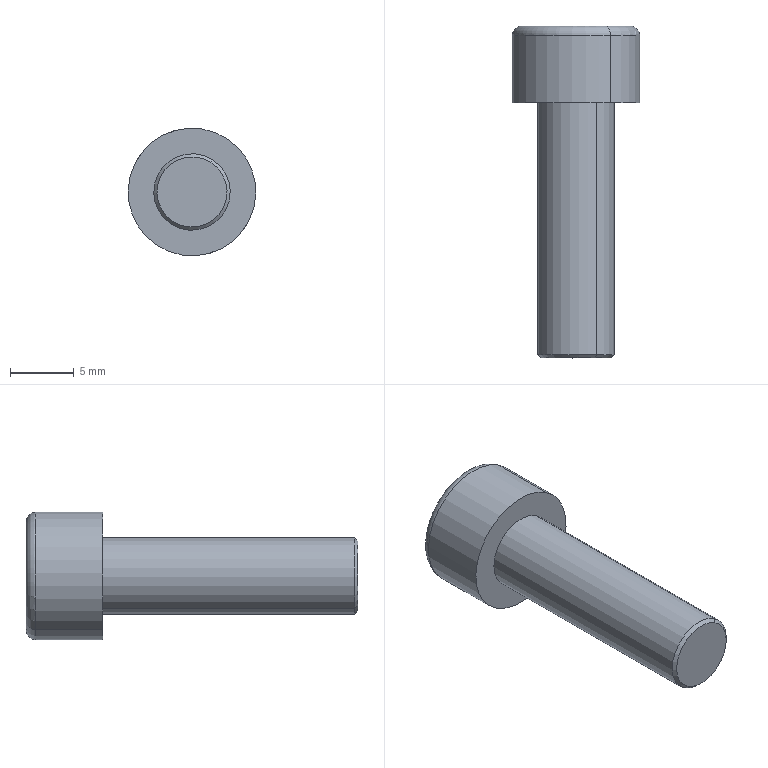Component | SolidWorks | hexagon socket head cap screws gb-17 | 1 solid | 25 faces | box 10 x 26 x 10 mm | volume 958 mm3 | plane 15 | cone 4 | cylinder 4 | torus 2 | commonest cylinder face diameters 6 x2 10 x2
STEP:
#1=COLOUR_RGB('',0.7922,0.8196,0.9333);
#2=FILL_AREA_STYLE_COLOUR('',#1);
#3=FILL_AREA_STYLE('',(#2));
#4=SURFACE_STYLE_FILL_AREA(#3);
#5=SURFACE_SIDE_STYLE('',(#4));
#6=SURFACE_STYLE_USAGE(.BOTH.,#5);
#7=PRESENTATION_STYLE_ASSIGNMENT((#6));
#8=CARTESIAN_POINT('',(-4.388,20.52,21.251));
#9=VERTEX_POINT('',#8);
#10=CARTESIAN_POINT('',(-4.271,20.52,21.433));
#11=VERTEX_POINT('',#10);
#12=CARTESIAN_POINT('',(-4.33,20.52,21.342));
#13=DIRECTION('',(0.,-1.,0.));
#14=DIRECTION('',(-0.5407,0.,-0.8412));
#15=AXIS2_PLACEMENT_3D('',#12,#13,#14);
#16=CIRCLE('',#15,0.1083);
#17=EDGE_CURVE('',#9,#11,#16,.T.);
#18=ORIENTED_EDGE('',*,*,#17,.F.);
#19=CARTESIAN_POINT('',(-4.394,20.53,21.243));
#20=VERTEX_POINT('',#19);
#21=CARTESIAN_POINT('',(-4.388,20.52,21.251));
#22=DIRECTION('',(-0.3823,0.7071,-0.5948));
#23=VECTOR('',#22,39.37);
#24=LINE('',#21,#23);
#25=EDGE_CURVE('',#9,#20,#24,.T.);
#26=ORIENTED_EDGE('',*,*,#25,.T.);
#27=CARTESIAN_POINT('',(-4.266,20.53,21.441));
#28=VERTEX_POINT('',#27);
#29=CARTESIAN_POINT('',(-4.33,20.53,21.342));
#30=DIRECTION('',(0.,1.,0.));
#31=DIRECTION('',(-0.5407,0.,-0.8412));
#32=AXIS2_PLACEMENT_3D('',#29,#30,#31);
#33=CIRCLE('',#32,0.1181);
#34=EDGE_CURVE('',#28,#20,#33,.T.);
#35=ORIENTED_EDGE('',*,*,#34,.F.);
#36=CARTESIAN_POINT('',(-4.271,20.52,21.433));
#37=DIRECTION('',(0.3823,0.7071,0.5948));
#38=VECTOR('',#37,39.37);
#39=LINE('',#36,#38);
#40=EDGE_CURVE('',#11,#28,#39,.T.);
#41=ORIENTED_EDGE('',*,*,#40,.F.);
#42=EDGE_LOOP('',(#18,#26,#35,#41));
#43=FACE_OUTER_BOUND('',#42,.T.);
#44=CARTESIAN_POINT('',(-4.33,20.52,21.342));
#45=DIRECTION('',(0.,1.,0.));
#46=DIRECTION('',(0.5407,0.,0.8412));
#47=AXIS2_PLACEMENT_3D('',#44,#45,#46);
#48=CONICAL_SURFACE('',#47,0.1083,0.7854);
#49=ADVANCED_FACE('',(#43),#48,.T.);
#50=CARTESIAN_POINT('',(-4.239,21.544,21.483));
#51=VERTEX_POINT('',#50);
#52=CARTESIAN_POINT('',(-4.42,21.544,21.201));
#53=VERTEX_POINT('',#52);
#54=CARTESIAN_POINT('',(-4.33,21.544,21.342));
#55=DIRECTION('',(0.,1.,0.));
#56=DIRECTION('',(-0.5407,0.,-0.8412));
#57=AXIS2_PLACEMENT_3D('',#54,#55,#56);
#58=CIRCLE('',#57,0.1673);
#59=EDGE_CURVE('',#51,#53,#58,.T.);
#60=ORIENTED_EDGE('',*,*,#59,.F.);
#61=CARTESIAN_POINT('',(-4.223,21.515,21.508));
#62=VERTEX_POINT('',#61);
#63=CARTESIAN_POINT('',(-4.239,21.515,21.483));
#64=DIRECTION('',(0.8412,0.,-0.5407));
#65=DIRECTION('',(-0.5407,0.,-0.8412));
#66=AXIS2_PLACEMENT_3D('',#63,#64,#65);
#67=CIRCLE('',#66,0.02953);
#68=EDGE_CURVE('',#51,#62,#67,.T.);
#69=ORIENTED_EDGE('',*,*,#68,.T.);
#70=CARTESIAN_POINT('',(-4.436,21.515,21.176));
#71=VERTEX_POINT('',#70);
#72=CARTESIAN_POINT('',(-4.33,21.515,21.342));
#73=DIRECTION('',(0.,-1.,0.));
#74=DIRECTION('',(-0.5407,0.,-0.8412));
#75=AXIS2_PLACEMENT_3D('',#72,#73,#74);
#76=CIRCLE('',#75,0.1969);
#77=EDGE_CURVE('',#71,#62,#76,.T.);
#78=ORIENTED_EDGE('',*,*,#77,.F.);
#79=CARTESIAN_POINT('',(-4.42,21.515,21.201));
#80=DIRECTION('',(-0.8412,0.,0.5407));
#81=DIRECTION('',(0.5407,0.,0.8412));
#82=AXIS2_PLACEMENT_3D('',#79,#80,#81);
#83=CIRCLE('',#82,0.02953);
#84=EDGE_CURVE('',#53,#71,#83,.T.);
#85=ORIENTED_EDGE('',*,*,#84,.F.);
#86=EDGE_LOOP('',(#60,#69,#78,#85));
#87=FACE_OUTER_BOUND('',#86,.T.);
#88=CARTESIAN_POINT('',(-4.33,21.515,21.342));
#89=DIRECTION('',(0.,-1.,0.));
#90=DIRECTION('',(-0.5407,0.,-0.8412));
#91=AXIS2_PLACEMENT_3D('',#88,#89,#90);
#92=TOROIDAL_SURFACE('',#91,0.1673,0.02953);
#93=ADVANCED_FACE('',(#87),#92,.T.);
#94=CARTESIAN_POINT('',(-4.33,21.369,21.342));
#95=VERTEX_POINT('',#94);
#96=CARTESIAN_POINT('',(-4.276,21.426,21.425));
#97=VERTEX_POINT('',#96);
#98=CARTESIAN_POINT('',(-4.276,21.426,21.425));
#99=DIRECTION('',(0.4682,0.5,0.7285));
#100=VECTOR('',#99,39.37);
#101=LINE('',#98,#100);
#102=EDGE_CURVE('',#95,#97,#101,.T.);
#103=ORIENTED_EDGE('',*,*,#102,.F.);
#104=CARTESIAN_POINT('',(-4.383,21.426,21.259));
#105=VERTEX_POINT('',#104);
#106=CARTESIAN_POINT('',(-4.383,21.426,21.259));
#107=DIRECTION('',(-0.4682,0.5,-0.7285));
#108=VECTOR('',#107,39.37);
#109=LINE('',#106,#108);
#110=EDGE_CURVE('',#95,#105,#109,.T.);
#111=ORIENTED_EDGE('',*,*,#110,.T.);
#112=CARTESIAN_POINT('',(-4.417,21.426,21.297));
#113=VERTEX_POINT('',#112);
#114=CARTESIAN_POINT('',(-4.33,21.426,21.342));
#115=DIRECTION('',(0.,1.,0.));
#116=DIRECTION('',(-0.5407,0.,-0.8412));
#117=AXIS2_PLACEMENT_3D('',#114,#115,#116);
#118=CIRCLE('',#117,0.09843);
#119=EDGE_CURVE('',#105,#113,#118,.T.);
#120=ORIENTED_EDGE('',*,*,#119,.T.);
#121=CARTESIAN_POINT('',(-4.413,21.426,21.395));
#122=VERTEX_POINT('',#121);
#123=CARTESIAN_POINT('',(-4.33,21.426,21.342));
#124=DIRECTION('',(0.,1.,0.));
#125=DIRECTION('',(-0.5407,0.,-0.8412));
#126=AXIS2_PLACEMENT_3D('',#123,#124,#125);
#127=CIRCLE('',#126,0.09843);
#128=EDGE_CURVE('',#113,#122,#127,.T.);
#129=ORIENTED_EDGE('',*,*,#128,.T.);
#130=CARTESIAN_POINT('',(-4.325,21.426,21.44));
#131=VERTEX_POINT('',#130);
#132=CARTESIAN_POINT('',(-4.33,21.426,21.342));
#133=DIRECTION('',(0.,1.,0.));
#134=DIRECTION('',(-0.5407,0.,-0.8412));
#135=AXIS2_PLACEMENT_3D('',#132,#133,#134);
#136=CIRCLE('',#135,0.09843);
#137=EDGE_CURVE('',#122,#131,#136,.T.);
#138=ORIENTED_EDGE('',*,*,#137,.T.);
#139=CARTESIAN_POINT('',(-4.33,21.426,21.342));
#140=DIRECTION('',(0.,1.,0.));
#141=DIRECTION('',(-0.5407,0.,-0.8412));
#142=AXIS2_PLACEMENT_3D('',#139,#140,#141);
#143=CIRCLE('',#142,0.09843);
#144=EDGE_CURVE('',#131,#97,#143,.T.);
#145=ORIENTED_EDGE('',*,*,#144,.T.);
#146=EDGE_LOOP('',(#103,#111,#120,#129,#138,#145));
#147=FACE_OUTER_BOUND('',#146,.T.);
#148=CARTESIAN_POINT('',(-4.33,21.426,21.342));
#149=DIRECTION('',(0.,1.,0.));
#150=DIRECTION('',(0.5407,0.,0.8412));
#151=AXIS2_PLACEMENT_3D('',#148,#149,#150);
#152=CONICAL_SURFACE('',#151,0.09843,1.047);
#153=ADVANCED_FACE('',(#147),#152,.F.);
#154=ORIENTED_EDGE('',*,*,#34,.T.);
#155=CARTESIAN_POINT('',(-4.394,21.308,21.243));
#156=VERTEX_POINT('',#155);
#157=CARTESIAN_POINT('',(-4.394,20.52,21.243));
#158=DIRECTION('',(0.,1.,0.));
#159=VECTOR('',#158,39.37);
#160=LINE('',#157,#159);
#161=EDGE_CURVE('',#20,#156,#160,.T.);
#162=ORIENTED_EDGE('',*,*,#161,.T.);
#163=CARTESIAN_POINT('',(-4.266,21.308,21.441));
#164=VERTEX_POINT('',#163);
#165=CARTESIAN_POINT('',(-4.33,21.308,21.342));
#166=DIRECTION('',(0.,-1.,0.));
#167=DIRECTION('',(-0.5407,0.,-0.8412));
#168=AXIS2_PLACEMENT_3D('',#165,#166,#167);
#169=CIRCLE('',#168,0.1181);
#170=EDGE_CURVE('',#156,#164,#169,.T.);
#171=ORIENTED_EDGE('',*,*,#170,.T.);
#172=CARTESIAN_POINT('',(-4.266,20.52,21.441));
#173=DIRECTION('',(0.,1.,0.));
#174=VECTOR('',#173,39.37);
#175=LINE('',#172,#174);
#176=EDGE_CURVE('',#28,#164,#175,.T.);
#177=ORIENTED_EDGE('',*,*,#176,.F.);
#178=EDGE_LOOP('',(#154,#162,#171,#177));
#179=FACE_OUTER_BOUND('',#178,.T.);
#180=CARTESIAN_POINT('',(-4.33,20.52,21.342));
#181=DIRECTION('',(0.,1.,0.));
#182=DIRECTION('',(0.5407,0.,0.8412));
#183=AXIS2_PLACEMENT_3D('',#180,#181,#182);
#184=CYLINDRICAL_SURFACE('',#183,0.1181);
#185=ADVANCED_FACE('',(#179),#184,.T.);
#186=CARTESIAN_POINT('',(-4.436,21.308,21.176));
#187=VERTEX_POINT('',#186);
#188=CARTESIAN_POINT('',(-4.223,21.308,21.508));
#189=VERTEX_POINT('',#188);
#190=CARTESIAN_POINT('',(-4.33,21.308,21.342));
#191=DIRECTION('',(0.,-1.,0.));
#192=DIRECTION('',(-0.5407,0.,-0.8412));
#193=AXIS2_PLACEMENT_3D('',#190,#191,#192);
#194=CIRCLE('',#193,0.1969);
#195=EDGE_CURVE('',#187,#189,#194,.T.);
#196=ORIENTED_EDGE('',*,*,#195,.F.);
#197=CARTESIAN_POINT('',(-4.436,21.308,21.176));
#198=DIRECTION('',(0.,1.,0.));
#199=VECTOR('',#198,39.37);
#200=LINE('',#197,#199);
#201=EDGE_CURVE('',#187,#71,#200,.T.);
#202=ORIENTED_EDGE('',*,*,#201,.T.);
#203=ORIENTED_EDGE('',*,*,#77,.T.);
#204=CARTESIAN_POINT('',(-4.223,21.308,21.508));
#205=DIRECTION('',(0.,1.,0.));
#206=VECTOR('',#205,39.37);
#207=LINE('',#204,#206);
#208=EDGE_CURVE('',#189,#62,#207,.T.);
#209=ORIENTED_EDGE('',*,*,#208,.F.);
#210=EDGE_LOOP('',(#196,#202,#203,#209));
#211=FACE_OUTER_BOUND('',#210,.T.);
#212=CARTESIAN_POINT('',(-4.33,21.308,21.342));
#213=DIRECTION('',(0.,1.,0.));
#214=DIRECTION('',(0.5407,0.,0.8412));
#215=AXIS2_PLACEMENT_3D('',#212,#213,#214);
#216=CYLINDRICAL_SURFACE('',#215,0.1969);
#217=ADVANCED_FACE('',(#211),#216,.T.);
#218=ORIENTED_EDGE('',*,*,#128,.F.);
#219=CARTESIAN_POINT('',(-4.443,21.426,21.347));
#220=VERTEX_POINT('',#219);
#221=CARTESIAN_POINT('',(-4.443,21.426,21.347));
#222=DIRECTION('',(0.4582,0.,-0.8888));
#223=VECTOR('',#222,39.37);
#224=LINE('',#221,#223);
#225=EDGE_CURVE('',#220,#113,#224,.T.);
#226=ORIENTED_EDGE('',*,*,#225,.F.);
#227=CARTESIAN_POINT('',(-4.382,21.426,21.443));
#228=DIRECTION('',(-0.5407,0.,-0.8412));
#229=VECTOR('',#228,39.37);
#230=LINE('',#227,#229);
#231=EDGE_CURVE('',#122,#220,#230,.T.);
#232=ORIENTED_EDGE('',*,*,#231,.F.);
#233=EDGE_LOOP('',(#218,#226,#232));
#234=FACE_OUTER_BOUND('',#233,.T.);
#235=CARTESIAN_POINT('',(-4.391,21.426,21.246));
#236=DIRECTION('',(0.,-1.,0.));
#237=DIRECTION('',(-0.5407,0.,-0.8412));
#238=AXIS2_PLACEMENT_3D('',#235,#236,#237);
#239=PLANE('',#238);
#240=ADVANCED_FACE('',(#234),#239,.F.);
#241=ORIENTED_EDGE('',*,*,#137,.F.);
#242=CARTESIAN_POINT('',(-4.382,21.426,21.443));
#243=VERTEX_POINT('',#242);
#244=CARTESIAN_POINT('',(-4.382,21.426,21.443));
#245=DIRECTION('',(-0.5407,0.,-0.8412));
#246=VECTOR('',#245,39.37);
#247=LINE('',#244,#246);
#248=EDGE_CURVE('',#243,#122,#247,.T.);
#249=ORIENTED_EDGE('',*,*,#248,.F.);
#250=CARTESIAN_POINT('',(-4.268,21.426,21.438));
#251=DIRECTION('',(-0.9989,0.,0.0476));
#252=VECTOR('',#251,39.37);
#253=LINE('',#250,#252);
#254=EDGE_CURVE('',#131,#243,#253,.T.);
#255=ORIENTED_EDGE('',*,*,#254,.F.);
#256=EDGE_LOOP('',(#241,#249,#255));
#257=FACE_OUTER_BOUND('',#256,.T.);
#258=CARTESIAN_POINT('',(-4.391,21.426,21.246));
#259=DIRECTION('',(0.,-1.,0.));
#260=DIRECTION('',(-0.5407,0.,-0.8412));
#261=AXIS2_PLACEMENT_3D('',#258,#259,#260);
#262=PLANE('',#261);
#263=ADVANCED_FACE('',(#257),#262,.F.);
#264=ORIENTED_EDGE('',*,*,#144,.F.);
#265=CARTESIAN_POINT('',(-4.268,21.426,21.438));
#266=VERTEX_POINT('',#265);
#267=CARTESIAN_POINT('',(-4.268,21.426,21.438));
#268=DIRECTION('',(-0.9989,0.,0.0476));
#269=VECTOR('',#268,39.37);
#270=LINE('',#267,#269);
#271=EDGE_CURVE('',#266,#131,#270,.T.);
#272=ORIENTED_EDGE('',*,*,#271,.F.);
#273=CARTESIAN_POINT('',(-4.242,21.426,21.387));
#274=VERTEX_POINT('',#273);
#275=CARTESIAN_POINT('',(-4.216,21.426,21.337));
#276=DIRECTION('',(-0.4582,0.,0.8888));
#277=VECTOR('',#276,39.37);
#278=LINE('',#275,#277);
#279=EDGE_CURVE('',#274,#266,#278,.T.);
#280=ORIENTED_EDGE('',*,*,#279,.F.);
#281=CARTESIAN_POINT('',(-4.33,21.426,21.342));
#282=DIRECTION('',(0.,1.,0.));
#283=DIRECTION('',(-0.5407,0.,-0.8412));
#284=AXIS2_PLACEMENT_3D('',#281,#282,#283);
#285=CIRCLE('',#284,0.09843);
#286=EDGE_CURVE('',#97,#274,#285,.T.);
#287=ORIENTED_EDGE('',*,*,#286,.F.);
#288=EDGE_LOOP('',(#264,#272,#280,#287));
#289=FACE_OUTER_BOUND('',#288,.T.);
#290=CARTESIAN_POINT('',(-4.391,21.426,21.246));
#291=DIRECTION('',(0.,-1.,0.));
#292=DIRECTION('',(-0.5407,0.,-0.8412));
#293=AXIS2_PLACEMENT_3D('',#290,#291,#292);
#294=PLANE('',#293);
#295=ADVANCED_FACE('',(#289),#294,.F.);
#296=CARTESIAN_POINT('',(-4.247,21.426,21.289));
#297=VERTEX_POINT('',#296);
#298=CARTESIAN_POINT('',(-4.33,21.426,21.342));
#299=DIRECTION('',(0.,1.,0.));
#300=DIRECTION('',(-0.5407,0.,-0.8412));
#301=AXIS2_PLACEMENT_3D('',#298,#299,#300);
#302=CIRCLE('',#301,0.09843);
#303=EDGE_CURVE('',#274,#297,#302,.T.);
#304=ORIENTED_EDGE('',*,*,#303,.F.);
#305=CARTESIAN_POINT('',(-4.216,21.426,21.337));
#306=VERTEX_POINT('',#305);
#307=CARTESIAN_POINT('',(-4.216,21.426,21.337));
#308=DIRECTION('',(-0.4582,0.,0.8888));
#309=VECTOR('',#308,39.37);
#310=LINE('',#307,#309);
#311=EDGE_CURVE('',#306,#274,#310,.T.);
#312=ORIENTED_EDGE('',*,*,#311,.F.);
#313=CARTESIAN_POINT('',(-4.278,21.426,21.241));
#314=DIRECTION('',(0.5407,0.,0.8412));
#315=VECTOR('',#314,39.37);
#316=LINE('',#313,#315);
#317=EDGE_CURVE('',#297,#306,#316,.T.);
#318=ORIENTED_EDGE('',*,*,#317,.F.);
#319=EDGE_LOOP('',(#304,#312,#318));
#320=FACE_OUTER_BOUND('',#319,.T.);
#321=CARTESIAN_POINT('',(-4.391,21.426,21.246));
#322=DIRECTION('',(0.,-1.,0.));
#323=DIRECTION('',(-0.5407,0.,-0.8412));
#324=AXIS2_PLACEMENT_3D('',#321,#322,#323);
#325=PLANE('',#324);
#326=ADVANCED_FACE('',(#320),#325,.F.);
#327=CARTESIAN_POINT('',(-4.334,21.426,21.244));
#328=VERTEX_POINT('',#327);
#329=CARTESIAN_POINT('',(-4.33,21.426,21.342));
#330=DIRECTION('',(0.,-1.,0.));
#331=DIRECTION('',(-0.5407,0.,-0.8412));
#332=AXIS2_PLACEMENT_3D('',#329,#330,#331);
#333=CIRCLE('',#332,0.09843);
#334=EDGE_CURVE('',#328,#297,#333,.T.);
#335=ORIENTED_EDGE('',*,*,#334,.T.);
#336=CARTESIAN_POINT('',(-4.278,21.426,21.241));
#337=VERTEX_POINT('',#336);
#338=CARTESIAN_POINT('',(-4.278,21.426,21.241));
#339=DIRECTION('',(0.5407,0.,0.8412));
#340=VECTOR('',#339,39.37);
#341=LINE('',#338,#340);
#342=EDGE_CURVE('',#337,#297,#341,.T.);
#343=ORIENTED_EDGE('',*,*,#342,.F.);
#344=CARTESIAN_POINT('',(-4.391,21.426,21.246));
#345=DIRECTION('',(0.9989,0.,-0.0476));
#346=VECTOR('',#345,39.37);
#347=LINE('',#344,#346);
#348=EDGE_CURVE('',#328,#337,#347,.T.);
#349=ORIENTED_EDGE('',*,*,#348,.F.);
#350=EDGE_LOOP('',(#335,#343,#349));
#351=FACE_OUTER_BOUND('',#350,.T.);
#352=CARTESIAN_POINT('',(-4.391,21.426,21.246));
#353=DIRECTION('',(0.,-1.,0.));
#354=DIRECTION('',(-0.5407,0.,-0.8412));
#355=AXIS2_PLACEMENT_3D('',#352,#353,#354);
#356=PLANE('',#355);
#357=ADVANCED_FACE('',(#351),#356,.F.);
#358=CARTESIAN_POINT('',(-4.33,21.426,21.342));
#359=DIRECTION('',(0.,1.,0.));
#360=DIRECTION('',(-0.5407,0.,-0.8412));
#361=AXIS2_PLACEMENT_3D('',#358,#359,#360);
#362=CIRCLE('',#361,0.09843);
#363=EDGE_CURVE('',#328,#105,#362,.T.);
#364=ORIENTED_EDGE('',*,*,#363,.F.);
#365=CARTESIAN_POINT('',(-4.391,21.426,21.246));
#366=VERTEX_POINT('',#365);
#367=CARTESIAN_POINT('',(-4.391,21.426,21.246));
#368=DIRECTION('',(0.9989,0.,-0.0476));
#369=VECTOR('',#368,39.37);
#370=LINE('',#367,#369);
#371=EDGE_CURVE('',#366,#328,#370,.T.);
#372=ORIENTED_EDGE('',*,*,#371,.F.);
#373=CARTESIAN_POINT('',(-4.443,21.426,21.347));
#374=DIRECTION('',(0.4582,0.,-0.8888));
#375=VECTOR('',#374,39.37);
#376=LINE('',#373,#375);
#377=EDGE_CURVE('',#113,#366,#376,.T.);
#378=ORIENTED_EDGE('',*,*,#377,.F.);
#379=ORIENTED_EDGE('',*,*,#119,.F.);
#380=EDGE_LOOP('',(#364,#372,#378,#379));
#381=FACE_OUTER_BOUND('',#380,.T.);
#382=CARTESIAN_POINT('',(-4.391,21.426,21.246));
#383=DIRECTION('',(0.,-1.,0.));
#384=DIRECTION('',(-0.5407,0.,-0.8412));
#385=AXIS2_PLACEMENT_3D('',#382,#383,#384);
#386=PLANE('',#385);
#387=ADVANCED_FACE('',(#381),#386,.F.);
#388=CARTESIAN_POINT('',(-4.33,21.544,21.342));
#389=DIRECTION('',(0.,1.,0.));
#390=DIRECTION('',(-0.5407,0.,-0.8412));
#391=AXIS2_PLACEMENT_3D('',#388,#389,#390);
#392=CIRCLE('',#391,0.1673);
#393=EDGE_CURVE('',#53,#51,#392,.T.);
#394=ORIENTED_EDGE('',*,*,#393,.T.);
#395=ORIENTED_EDGE('',*,*,#59,.T.);
#396=EDGE_LOOP('',(#394,#395));
#397=FACE_OUTER_BOUND('',#396,.T.);
#398=CARTESIAN_POINT('',(-4.443,21.544,21.347));
#399=VERTEX_POINT('',#398);
#400=CARTESIAN_POINT('',(-4.391,21.544,21.246));
#401=VERTEX_POINT('',#400);
#402=CARTESIAN_POINT('',(-4.443,21.544,21.347));
#403=DIRECTION('',(0.4582,0.,-0.8888));
#404=VECTOR('',#403,39.37);
#405=LINE('',#402,#404);
#406=EDGE_CURVE('',#399,#401,#405,.T.);
#407=ORIENTED_EDGE('',*,*,#406,.T.);
#408=CARTESIAN_POINT('',(-4.278,21.544,21.241));
#409=VERTEX_POINT('',#408);
#410=CARTESIAN_POINT('',(-4.391,21.544,21.246));
#411=DIRECTION('',(0.9989,0.,-0.0476));
#412=VECTOR('',#411,39.37);
#413=LINE('',#410,#412);
#414=EDGE_CURVE('',#401,#409,#413,.T.);
#415=ORIENTED_EDGE('',*,*,#414,.T.);
#416=CARTESIAN_POINT('',(-4.216,21.544,21.337));
#417=VERTEX_POINT('',#416);
#418=CARTESIAN_POINT('',(-4.278,21.544,21.241));
#419=DIRECTION('',(0.5407,0.,0.8412));
#420=VECTOR('',#419,39.37);
#421=LINE('',#418,#420);
#422=EDGE_CURVE('',#409,#417,#421,.T.);
#423=ORIENTED_EDGE('',*,*,#422,.T.);
#424=CARTESIAN_POINT('',(-4.268,21.544,21.438));
#425=VERTEX_POINT('',#424);
#426=CARTESIAN_POINT('',(-4.216,21.544,21.337));
#427=DIRECTION('',(-0.4582,0.,0.8888));
#428=VECTOR('',#427,39.37);
#429=LINE('',#426,#428);
#430=EDGE_CURVE('',#417,#425,#429,.T.);
#431=ORIENTED_EDGE('',*,*,#430,.T.);
#432=CARTESIAN_POINT('',(-4.382,21.544,21.443));
#433=VERTEX_POINT('',#432);
#434=CARTESIAN_POINT('',(-4.268,21.544,21.438));
#435=DIRECTION('',(-0.9989,0.,0.0476));
#436=VECTOR('',#435,39.37);
#437=LINE('',#434,#436);
#438=EDGE_CURVE('',#425,#433,#437,.T.);
#439=ORIENTED_EDGE('',*,*,#438,.T.);
#440=CARTESIAN_POINT('',(-4.382,21.544,21.443));
#441=DIRECTION('',(-0.5407,0.,-0.8412));
#442=VECTOR('',#441,39.37);
#443=LINE('',#440,#442);
#444=EDGE_CURVE('',#433,#399,#443,.T.);
#445=ORIENTED_EDGE('',*,*,#444,.T.);
#446=EDGE_LOOP('',(#407,#415,#423,#431,#439,#445));
#447=FACE_BOUND('',#446,.T.);
#448=CARTESIAN_POINT('',(-4.33,21.544,21.342));
#449=DIRECTION('',(0.,-1.,0.));
#450=DIRECTION('',(-0.5407,0.,-0.8412));
#451=AXIS2_PLACEMENT_3D('',#448,#449,#450);
#452=PLANE('',#451);
#453=ADVANCED_FACE('',(#397,#447),#452,.F.);
#454=CARTESIAN_POINT('',(-4.33,21.308,21.342));
#455=DIRECTION('',(0.,-1.,0.));
#456=DIRECTION('',(-0.5407,0.,-0.8412));
#457=AXIS2_PLACEMENT_3D('',#454,#455,#456);
#458=CIRCLE('',#457,0.1969);
#459=EDGE_CURVE('',#189,#187,#458,.T.);
#460=ORIENTED_EDGE('',*,*,#459,.T.);
#461=ORIENTED_EDGE('',*,*,#195,.T.);
#462=EDGE_LOOP('',(#460,#461));
#463=FACE_OUTER_BOUND('',#462,.T.);
#464=CARTESIAN_POINT('',(-4.33,21.308,21.342));
#465=DIRECTION('',(0.,-1.,0.));
#466=DIRECTION('',(-0.5407,0.,-0.8412));
#467=AXIS2_PLACEMENT_3D('',#464,#465,#466);
#468=CIRCLE('',#467,0.1181);
#469=EDGE_CURVE('',#164,#156,#468,.T.);
#470=ORIENTED_EDGE('',*,*,#469,.F.);
#471=ORIENTED_EDGE('',*,*,#170,.F.);
#472=EDGE_LOOP('',(#470,#471));
#473=FACE_BOUND('',#472,.T.);
#474=CARTESIAN_POINT('',(-4.33,21.308,21.342));
#475=DIRECTION('',(0.,-1.,0.));
#476=DIRECTION('',(-0.5407,0.,-0.8412));
#477=AXIS2_PLACEMENT_3D('',#474,#475,#476);
#478=PLANE('',#477);
#479=ADVANCED_FACE('',(#463,#473),#478,.T.);
#480=ORIENTED_EDGE('',*,*,#201,.F.);
#481=ORIENTED_EDGE('',*,*,#459,.F.);
#482=ORIENTED_EDGE('',*,*,#208,.T.);
#483=CARTESIAN_POINT('',(-4.33,21.515,21.342));
#484=DIRECTION('',(0.,-1.,0.));
#485=DIRECTION('',(-0.5407,0.,-0.8412));
#486=AXIS2_PLACEMENT_3D('',#483,#484,#485);
#487=CIRCLE('',#486,0.1969);
#488=EDGE_CURVE('',#62,#71,#487,.T.);
#489=ORIENTED_EDGE('',*,*,#488,.T.);
#490=EDGE_LOOP('',(#480,#481,#482,#489));
#491=FACE_OUTER_BOUND('',#490,.T.);
#492=CARTESIAN_POINT('',(-4.33,21.308,21.342));
#493=DIRECTION('',(0.,1.,0.));
#494=DIRECTION('',(0.5407,0.,0.8412));
#495=AXIS2_PLACEMENT_3D('',#492,#493,#494);
#496=CYLINDRICAL_SURFACE('',#495,0.1969);
#497=ADVANCED_FACE('',(#491),#496,.T.);
#498=ORIENTED_EDGE('',*,*,#161,.F.);
#499=CARTESIAN_POINT('',(-4.33,20.53,21.342));
#500=DIRECTION('',(0.,1.,0.));
#501=DIRECTION('',(-0.5407,0.,-0.8412));
#502=AXIS2_PLACEMENT_3D('',#499,#500,#501);
#503=CIRCLE('',#502,0.1181);
#504=EDGE_CURVE('',#20,#28,#503,.T.);
#505=ORIENTED_EDGE('',*,*,#504,.T.);
#506=ORIENTED_EDGE('',*,*,#176,.T.);
#507=ORIENTED_EDGE('',*,*,#469,.T.);
#508=EDGE_LOOP('',(#498,#505,#506,#507));
#509=FACE_OUTER_BOUND('',#508,.T.);
#510=CARTESIAN_POINT('',(-4.33,20.52,21.342));
#511=DIRECTION('',(0.,1.,0.));
#512=DIRECTION('',(0.5407,0.,0.8412));
#513=AXIS2_PLACEMENT_3D('',#510,#511,#512);
#514=CYLINDRICAL_SURFACE('',#513,0.1181);
#515=ADVANCED_FACE('',(#509),#514,.T.);
#516=CARTESIAN_POINT('',(-4.33,20.52,21.342));
#517=DIRECTION('',(0.,-1.,0.));
#518=DIRECTION('',(-0.5407,0.,-0.8412));
#519=AXIS2_PLACEMENT_3D('',#516,#517,#518);
#520=CIRCLE('',#519,0.1083);
#521=EDGE_CURVE('',#11,#9,#520,.T.);
#522=ORIENTED_EDGE('',*,*,#521,.T.);
#523=ORIENTED_EDGE('',*,*,#17,.T.);
#524=EDGE_LOOP('',(#522,#523));
#525=FACE_OUTER_BOUND('',#524,.T.);
#526=CARTESIAN_POINT('',(-4.33,20.52,21.342));
#527=DIRECTION('',(0.,-1.,0.));
#528=DIRECTION('',(-0.5407,0.,-0.8412));
#529=AXIS2_PLACEMENT_3D('',#526,#527,#528);
#530=PLANE('',#529);
#531=ADVANCED_FACE('',(#525),#530,.T.);
#532=ORIENTED_EDGE('',*,*,#406,.F.);
#533=CARTESIAN_POINT('',(-4.443,21.426,21.347));
#534=DIRECTION('',(0.,1.,0.));
#535=VECTOR('',#534,39.37);
#536=LINE('',#533,#535);
#537=EDGE_CURVE('',#220,#399,#536,.T.);
#538=ORIENTED_EDGE('',*,*,#537,.F.);
#539=ORIENTED_EDGE('',*,*,#225,.T.);
#540=ORIENTED_EDGE('',*,*,#377,.T.);
#541=CARTESIAN_POINT('',(-4.391,21.426,21.246));
#542=DIRECTION('',(0.,1.,0.));
#543=VECTOR('',#542,39.37);
#544=LINE('',#541,#543);
#545=EDGE_CURVE('',#366,#401,#544,.T.);
#546=ORIENTED_EDGE('',*,*,#545,.T.);
#547=EDGE_LOOP('',(#532,#538,#539,#540,#546));
#548=FACE_OUTER_BOUND('',#547,.T.);
#549=CARTESIAN_POINT('',(-4.443,21.426,21.347));
#550=DIRECTION('',(0.8888,0.,0.4582));
#551=DIRECTION('',(-0.4582,0.,0.8888));
#552=AXIS2_PLACEMENT_3D('',#549,#550,#551);
#553=PLANE('',#552);
#554=ADVANCED_FACE('',(#548),#553,.T.);
#555=ORIENTED_EDGE('',*,*,#414,.F.);
#556=ORIENTED_EDGE('',*,*,#545,.F.);
#557=ORIENTED_EDGE('',*,*,#371,.T.);
#558=ORIENTED_EDGE('',*,*,#348,.T.);
#559=CARTESIAN_POINT('',(-4.278,21.426,21.241));
#560=DIRECTION('',(0.,1.,0.));
#561=VECTOR('',#560,39.37);
#562=LINE('',#559,#561);
#563=EDGE_CURVE('',#337,#409,#562,.T.);
#564=ORIENTED_EDGE('',*,*,#563,.T.);
#565=EDGE_LOOP('',(#555,#556,#557,#558,#564));
#566=FACE_OUTER_BOUND('',#565,.T.);
#567=CARTESIAN_POINT('',(-4.391,21.426,21.246));
#568=DIRECTION('',(0.0476,0.,0.9989));
#569=DIRECTION('',(-0.9989,0.,0.0476));
#570=AXIS2_PLACEMENT_3D('',#567,#568,#569);
#571=PLANE('',#570);
#572=ADVANCED_FACE('',(#566),#571,.T.);
#573=ORIENTED_EDGE('',*,*,#422,.F.);
#574=ORIENTED_EDGE('',*,*,#563,.F.);
#575=ORIENTED_EDGE('',*,*,#342,.T.);
#576=ORIENTED_EDGE('',*,*,#317,.T.);
#577=CARTESIAN_POINT('',(-4.216,21.426,21.337));
#578=DIRECTION('',(0.,1.,0.));
#579=VECTOR('',#578,39.37);
#580=LINE('',#577,#579);
#581=EDGE_CURVE('',#306,#417,#580,.T.);
#582=ORIENTED_EDGE('',*,*,#581,.T.);
#583=EDGE_LOOP('',(#573,#574,#575,#576,#582));
#584=FACE_OUTER_BOUND('',#583,.T.);
#585=CARTESIAN_POINT('',(-4.278,21.426,21.241));
#586=DIRECTION('',(-0.8412,0.,0.5407));
#587=DIRECTION('',(-0.5407,0.,-0.8412));
#588=AXIS2_PLACEMENT_3D('',#585,#586,#587);
#589=PLANE('',#588);
#590=ADVANCED_FACE('',(#584),#589,.T.);
#591=ORIENTED_EDGE('',*,*,#430,.F.);
#592=ORIENTED_EDGE('',*,*,#581,.F.);
#593=ORIENTED_EDGE('',*,*,#311,.T.);
#594=ORIENTED_EDGE('',*,*,#279,.T.);
#595=CARTESIAN_POINT('',(-4.268,21.426,21.438));
#596=DIRECTION('',(0.,1.,0.));
#597=VECTOR('',#596,39.37);
#598=LINE('',#595,#597);
#599=EDGE_CURVE('',#266,#425,#598,.T.);
#600=ORIENTED_EDGE('',*,*,#599,.T.);
#601=EDGE_LOOP('',(#591,#592,#593,#594,#600));
#602=FACE_OUTER_BOUND('',#601,.T.);
#603=CARTESIAN_POINT('',(-4.216,21.426,21.337));
#604=DIRECTION('',(-0.8888,0.,-0.4582));
#605=DIRECTION('',(0.4582,0.,-0.8888));
#606=AXIS2_PLACEMENT_3D('',#603,#604,#605);
#607=PLANE('',#606);
#608=ADVANCED_FACE('',(#602),#607,.T.);
#609=ORIENTED_EDGE('',*,*,#438,.F.);
#610=ORIENTED_EDGE('',*,*,#599,.F.);
#611=ORIENTED_EDGE('',*,*,#271,.T.);
#612=ORIENTED_EDGE('',*,*,#254,.T.);
#613=CARTESIAN_POINT('',(-4.382,21.426,21.443));
#614=DIRECTION('',(0.,1.,0.));
#615=VECTOR('',#614,39.37);
#616=LINE('',#613,#615);
#617=EDGE_CURVE('',#243,#433,#616,.T.);
#618=ORIENTED_EDGE('',*,*,#617,.T.);
#619=EDGE_LOOP('',(#609,#610,#611,#612,#618));
#620=FACE_OUTER_BOUND('',#619,.T.);
#621=CARTESIAN_POINT('',(-4.268,21.426,21.438));
#622=DIRECTION('',(-0.0476,0.,-0.9989));
#623=DIRECTION('',(0.9989,0.,-0.0476));
#624=AXIS2_PLACEMENT_3D('',#621,#622,#623);
#625=PLANE('',#624);
#626=ADVANCED_FACE('',(#620),#625,.T.);
#627=ORIENTED_EDGE('',*,*,#444,.F.);
#628=ORIENTED_EDGE('',*,*,#617,.F.);
#629=ORIENTED_EDGE('',*,*,#248,.T.);
#630=ORIENTED_EDGE('',*,*,#231,.T.);
#631=ORIENTED_EDGE('',*,*,#537,.T.);
#632=EDGE_LOOP('',(#627,#628,#629,#630,#631));
#633=FACE_OUTER_BOUND('',#632,.T.);
#634=CARTESIAN_POINT('',(-4.382,21.426,21.443));
#635=DIRECTION('',(0.8412,0.,-0.5407));
#636=DIRECTION('',(0.5407,0.,0.8412));
#637=AXIS2_PLACEMENT_3D('',#634,#635,#636);
#638=PLANE('',#637);
#639=ADVANCED_FACE('',(#633),#638,.T.);
#640=ORIENTED_EDGE('',*,*,#110,.F.);
#641=ORIENTED_EDGE('',*,*,#102,.T.);
#642=ORIENTED_EDGE('',*,*,#286,.T.);
#643=ORIENTED_EDGE('',*,*,#303,.T.);
#644=ORIENTED_EDGE('',*,*,#334,.F.);
#645=ORIENTED_EDGE('',*,*,#363,.T.);
#646=EDGE_LOOP('',(#640,#641,#642,#643,#644,#645));
#647=FACE_OUTER_BOUND('',#646,.T.);
#648=CARTESIAN_POINT('',(-4.33,21.426,21.342));
#649=DIRECTION('',(0.,1.,0.));
#650=DIRECTION('',(0.5407,0.,0.8412));
#651=AXIS2_PLACEMENT_3D('',#648,#649,#650);
#652=CONICAL_SURFACE('',#651,0.09843,1.047);
#653=ADVANCED_FACE('',(#647),#652,.F.);
#654=ORIENTED_EDGE('',*,*,#68,.F.);
#655=ORIENTED_EDGE('',*,*,#393,.F.);
#656=ORIENTED_EDGE('',*,*,#84,.T.);
#657=ORIENTED_EDGE('',*,*,#488,.F.);
#658=EDGE_LOOP('',(#654,#655,#656,#657));
#659=FACE_OUTER_BOUND('',#658,.T.);
#660=CARTESIAN_POINT('',(-4.33,21.515,21.342));
#661=DIRECTION('',(0.,-1.,0.));
#662=DIRECTION('',(-0.5407,0.,-0.8412));
#663=AXIS2_PLACEMENT_3D('',#660,#661,#662);
#664=TOROIDAL_SURFACE('',#663,0.1673,0.02953);
#665=ADVANCED_FACE('',(#659),#664,.T.);
#666=ORIENTED_EDGE('',*,*,#25,.F.);
#667=ORIENTED_EDGE('',*,*,#521,.F.);
#668=ORIENTED_EDGE('',*,*,#40,.T.);
#669=ORIENTED_EDGE('',*,*,#504,.F.);
#670=EDGE_LOOP('',(#666,#667,#668,#669));
#671=FACE_OUTER_BOUND('',#670,.T.);
#672=CARTESIAN_POINT('',(-4.33,20.52,21.342));
#673=DIRECTION('',(0.,1.,0.));
#674=DIRECTION('',(0.5407,0.,0.8412));
#675=AXIS2_PLACEMENT_3D('',#672,#673,#674);
#676=CONICAL_SURFACE('',#675,0.1083,0.7854);
#677=ADVANCED_FACE('',(#671),#676,.T.);
#678=CLOSED_SHELL('',(#49,#93,#153,#185,#217,#240,#263,#295,#326,#357,#387,#453,#479,#497,#515,#531,#554,#572,#590,#608,#626,#639,#653,#665,#677));
#679=MANIFOLD_SOLID_BREP('',#678);
#680=STYLED_ITEM('',(#7),#679);
#681=(LENGTH_UNIT()NAMED_UNIT(*)SI_UNIT($,.METRE.));
#682=LENGTH_MEASURE_WITH_UNIT(LENGTH_MEASURE(0.0254),#681);
#683=DIMENSIONAL_EXPONENTS(1.,0.,0.,0.,0.,0.,0.);
#684=(CONVERSION_BASED_UNIT('',#682)LENGTH_UNIT()NAMED_UNIT(#683));
#685=UNCERTAINTY_MEASURE_WITH_UNIT(LENGTH_MEASURE(0.00001),#684,'','');
#686=(NAMED_UNIT(*)PLANE_ANGLE_UNIT()SI_UNIT($,.RADIAN.));
#687=(NAMED_UNIT(*)SI_UNIT($,.STERADIAN.)SOLID_ANGLE_UNIT());
#688=(GEOMETRIC_REPRESENTATION_CONTEXT(3)GLOBAL_UNCERTAINTY_ASSIGNED_CONTEXT((#685))GLOBAL_UNIT_ASSIGNED_CONTEXT((#684,#686,#687))REPRESENTATION_CONTEXT('',''));
#689=MECHANICAL_DESIGN_GEOMETRIC_PRESENTATION_REPRESENTATION('',(#680),#688);
#690=PRESENTATION_LAYER_ASSIGNMENT('','',(#680));
#691=CARTESIAN_POINT('',(0.,0.,0.));
#692=DIRECTION('',(0.,0.,1.));
#693=DIRECTION('',(1.,0.,0.));
#694=AXIS2_PLACEMENT_3D('',#691,#692,#693);
#695=(LENGTH_UNIT()NAMED_UNIT(*)SI_UNIT($,.METRE.));
#696=LENGTH_MEASURE_WITH_UNIT(LENGTH_MEASURE(0.0254),#695);
#697=DIMENSIONAL_EXPONENTS(1.,0.,0.,0.,0.,0.,0.);
#698=(CONVERSION_BASED_UNIT('',#696)LENGTH_UNIT()NAMED_UNIT(#697));
#699=UNCERTAINTY_MEASURE_WITH_UNIT(LENGTH_MEASURE(0.00001),#698,'','');
#700=(NAMED_UNIT(*)PLANE_ANGLE_UNIT()SI_UNIT($,.RADIAN.));
#701=(NAMED_UNIT(*)SI_UNIT($,.STERADIAN.)SOLID_ANGLE_UNIT());
#702=(GEOMETRIC_REPRESENTATION_CONTEXT(3)GLOBAL_UNCERTAINTY_ASSIGNED_CONTEXT((#699))GLOBAL_UNIT_ASSIGNED_CONTEXT((#698,#700,#701))REPRESENTATION_CONTEXT('',''));
#703=ADVANCED_BREP_SHAPE_REPRESENTATION('',(#679,#694),#702);